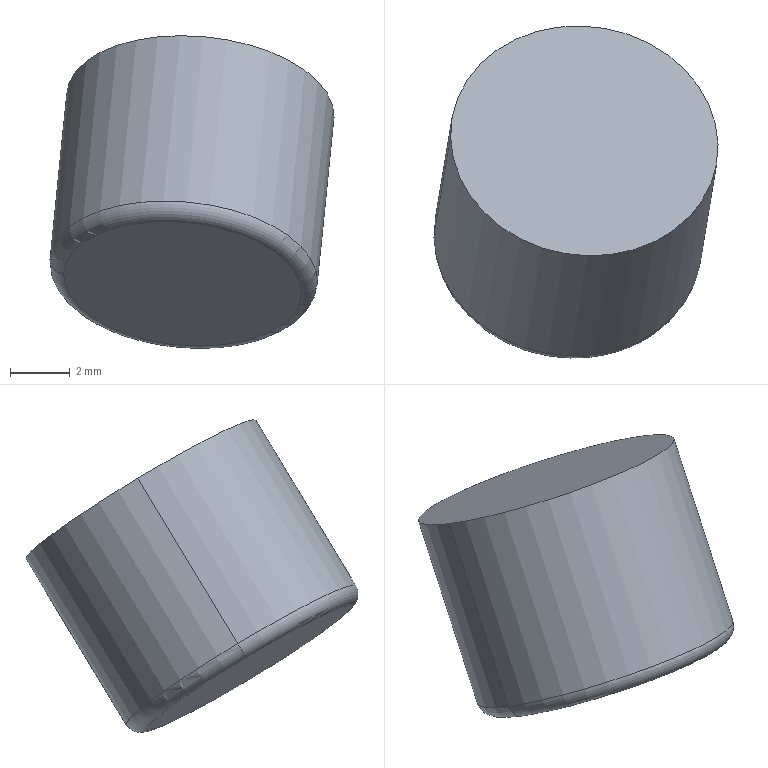Component | SolidWorks | 14AC-24-1-015-1 | 1 solid | 6 faces | box 9.53 x 11.13 x 10.48 mm | volume 444 mm3 | torus 2 | cylinder 2 | plane 2 | commonest cylinder face diameters 9 x2
build123d program:
from build123d import *

# Parameters (mm, degrees)
SKETCH1_R           = 4.5
BOSS_EXTRUDE1_DEPTH = 7
FILLET1_R           = 0.5


with BuildPart() as part:
    # Sketch1 → Boss-Extrude1 (new body)
    with BuildSketch(Plane.XY):
        Circle(SKETCH1_R)
    extrude(amount=BOSS_EXTRUDE1_DEPTH)

    # Fillet1
    fillet1_edges = [part.edges().sort_by_distance(p)[0] for p in [
        (-4.5, 0, 0),
    ]]
    fillet(fillet1_edges, radius=FILLET1_R)


solid = part.part

# Placed as in the assembly
solid = solid.moved(Location((420.449, -136.308, -150.512), (-31.129, 4.92, 15.941)))
STEP:
#1=COLOUR_RGB('',0.7922,0.8196,0.9333);
#2=FILL_AREA_STYLE_COLOUR('',#1);
#3=FILL_AREA_STYLE('',(#2));
#4=SURFACE_STYLE_FILL_AREA(#3);
#5=SURFACE_SIDE_STYLE('',(#4));
#6=SURFACE_STYLE_USAGE(.BOTH.,#5);
#7=PRESENTATION_STYLE_ASSIGNMENT((#6));
#8=CARTESIAN_POINT('',(16.396,-5.363,-5.912));
#9=VERTEX_POINT('',#8);
#10=CARTESIAN_POINT('',(16.71,-5.37,-5.939));
#11=VERTEX_POINT('',#10);
#12=CARTESIAN_POINT('',(16.553,-5.366,-5.926));
#13=DIRECTION('',(-0.08576,-0.5151,-0.8529));
#14=DIRECTION('',(0.996,-0.02384,-0.08576));
#15=AXIS2_PLACEMENT_3D('',#12,#13,#14);
#16=CIRCLE('',#15,0.1575);
#17=EDGE_CURVE('',#9,#11,#16,.T.);
#18=ORIENTED_EDGE('',*,*,#17,.F.);
#19=CARTESIAN_POINT('',(16.378,-5.352,-5.894));
#20=VERTEX_POINT('',#19);
#21=CARTESIAN_POINT('',(16.398,-5.353,-5.895));
#22=DIRECTION('',(-0.02384,0.8568,-0.5151));
#23=DIRECTION('',(0.,0.5152,0.8571));
#24=AXIS2_PLACEMENT_3D('',#21,#22,#23);
#25=CIRCLE('',#24,0.01969);
#26=EDGE_CURVE('',#9,#20,#25,.T.);
#27=ORIENTED_EDGE('',*,*,#26,.T.);
#28=CARTESIAN_POINT('',(16.731,-5.361,-5.924));
#29=VERTEX_POINT('',#28);
#30=CARTESIAN_POINT('',(16.555,-5.356,-5.909));
#31=DIRECTION('',(0.08576,0.5151,0.8529));
#32=DIRECTION('',(0.996,-0.02384,-0.08576));
#33=AXIS2_PLACEMENT_3D('',#30,#31,#32);
#34=CIRCLE('',#33,0.1772);
#35=EDGE_CURVE('',#29,#20,#34,.T.);
#36=ORIENTED_EDGE('',*,*,#35,.F.);
#37=CARTESIAN_POINT('',(16.712,-5.36,-5.922));
#38=DIRECTION('',(0.02384,-0.8568,0.5151));
#39=DIRECTION('',(0.,-0.5152,-0.8571));
#40=AXIS2_PLACEMENT_3D('',#37,#38,#39);
#41=CIRCLE('',#40,0.01969);
#42=EDGE_CURVE('',#11,#29,#41,.T.);
#43=ORIENTED_EDGE('',*,*,#42,.F.);
#44=EDGE_LOOP('',(#18,#27,#36,#43));
#45=FACE_OUTER_BOUND('',#44,.T.);
#46=CARTESIAN_POINT('',(16.555,-5.356,-5.909));
#47=DIRECTION('',(0.08576,0.5151,0.8529));
#48=DIRECTION('',(0.996,-0.02384,-0.08576));
#49=AXIS2_PLACEMENT_3D('',#46,#47,#48);
#50=TOROIDAL_SURFACE('',#49,0.1575,0.01969);
#51=ADVANCED_FACE('',(#45),#50,.T.);
#52=CARTESIAN_POINT('',(16.753,-5.229,-5.706));
#53=VERTEX_POINT('',#52);
#54=CARTESIAN_POINT('',(16.4,-5.22,-5.675));
#55=VERTEX_POINT('',#54);
#56=CARTESIAN_POINT('',(16.577,-5.224,-5.691));
#57=DIRECTION('',(0.08576,0.5151,0.8529));
#58=DIRECTION('',(0.996,-0.02384,-0.08576));
#59=AXIS2_PLACEMENT_3D('',#56,#57,#58);
#60=CIRCLE('',#59,0.1772);
#61=EDGE_CURVE('',#53,#55,#60,.T.);
#62=ORIENTED_EDGE('',*,*,#61,.F.);
#63=CARTESIAN_POINT('',(16.753,-5.229,-5.706));
#64=DIRECTION('',(-0.08576,-0.5151,-0.8529));
#65=VECTOR('',#64,39.37);
#66=LINE('',#63,#65);
#67=EDGE_CURVE('',#53,#29,#66,.T.);
#68=ORIENTED_EDGE('',*,*,#67,.T.);
#69=ORIENTED_EDGE('',*,*,#35,.T.);
#70=CARTESIAN_POINT('',(16.4,-5.22,-5.675));
#71=DIRECTION('',(-0.08576,-0.5151,-0.8529));
#72=VECTOR('',#71,39.37);
#73=LINE('',#70,#72);
#74=EDGE_CURVE('',#55,#20,#73,.T.);
#75=ORIENTED_EDGE('',*,*,#74,.F.);
#76=EDGE_LOOP('',(#62,#68,#69,#75));
#77=FACE_OUTER_BOUND('',#76,.T.);
#78=CARTESIAN_POINT('',(16.577,-5.224,-5.691));
#79=DIRECTION('',(-0.08576,-0.5151,-0.8529));
#80=DIRECTION('',(-0.996,0.02384,0.08576));
#81=AXIS2_PLACEMENT_3D('',#78,#79,#80);
#82=CYLINDRICAL_SURFACE('',#81,0.1772);
#83=ADVANCED_FACE('',(#77),#82,.T.);
#84=ORIENTED_EDGE('',*,*,#67,.F.);
#85=CARTESIAN_POINT('',(16.577,-5.224,-5.691));
#86=DIRECTION('',(0.08576,0.5151,0.8529));
#87=DIRECTION('',(0.996,-0.02384,-0.08576));
#88=AXIS2_PLACEMENT_3D('',#85,#86,#87);
#89=CIRCLE('',#88,0.1772);
#90=EDGE_CURVE('',#55,#53,#89,.T.);
#91=ORIENTED_EDGE('',*,*,#90,.F.);
#92=ORIENTED_EDGE('',*,*,#74,.T.);
#93=CARTESIAN_POINT('',(16.555,-5.356,-5.909));
#94=DIRECTION('',(0.08576,0.5151,0.8529));
#95=DIRECTION('',(0.996,-0.02384,-0.08576));
#96=AXIS2_PLACEMENT_3D('',#93,#94,#95);
#97=CIRCLE('',#96,0.1772);
#98=EDGE_CURVE('',#20,#29,#97,.T.);
#99=ORIENTED_EDGE('',*,*,#98,.T.);
#100=EDGE_LOOP('',(#84,#91,#92,#99));
#101=FACE_OUTER_BOUND('',#100,.T.);
#102=CARTESIAN_POINT('',(16.577,-5.224,-5.691));
#103=DIRECTION('',(-0.08576,-0.5151,-0.8529));
#104=DIRECTION('',(-0.996,0.02384,0.08576));
#105=AXIS2_PLACEMENT_3D('',#102,#103,#104);
#106=CYLINDRICAL_SURFACE('',#105,0.1772);
#107=ADVANCED_FACE('',(#101),#106,.T.);
#108=ORIENTED_EDGE('',*,*,#90,.T.);
#109=ORIENTED_EDGE('',*,*,#61,.T.);
#110=EDGE_LOOP('',(#108,#109));
#111=FACE_OUTER_BOUND('',#110,.T.);
#112=CARTESIAN_POINT('',(16.577,-5.224,-5.691));
#113=DIRECTION('',(0.08576,0.5151,0.8529));
#114=DIRECTION('',(0.996,-0.02384,-0.08576));
#115=AXIS2_PLACEMENT_3D('',#112,#113,#114);
#116=PLANE('',#115);
#117=ADVANCED_FACE('',(#111),#116,.T.);
#118=CARTESIAN_POINT('',(16.553,-5.366,-5.926));
#119=DIRECTION('',(-0.08576,-0.5151,-0.8529));
#120=DIRECTION('',(0.996,-0.02384,-0.08576));
#121=AXIS2_PLACEMENT_3D('',#118,#119,#120);
#122=CIRCLE('',#121,0.1575);
#123=EDGE_CURVE('',#11,#9,#122,.T.);
#124=ORIENTED_EDGE('',*,*,#123,.T.);
#125=ORIENTED_EDGE('',*,*,#17,.T.);
#126=EDGE_LOOP('',(#124,#125));
#127=FACE_OUTER_BOUND('',#126,.T.);
#128=CARTESIAN_POINT('',(16.553,-5.366,-5.926));
#129=DIRECTION('',(0.08576,0.5151,0.8529));
#130=DIRECTION('',(0.996,-0.02384,-0.08576));
#131=AXIS2_PLACEMENT_3D('',#128,#129,#130);
#132=PLANE('',#131);
#133=ADVANCED_FACE('',(#127),#132,.F.);
#134=ORIENTED_EDGE('',*,*,#26,.F.);
#135=ORIENTED_EDGE('',*,*,#123,.F.);
#136=ORIENTED_EDGE('',*,*,#42,.T.);
#137=ORIENTED_EDGE('',*,*,#98,.F.);
#138=EDGE_LOOP('',(#134,#135,#136,#137));
#139=FACE_OUTER_BOUND('',#138,.T.);
#140=CARTESIAN_POINT('',(16.555,-5.356,-5.909));
#141=DIRECTION('',(0.08576,0.5151,0.8529));
#142=DIRECTION('',(0.996,-0.02384,-0.08576));
#143=AXIS2_PLACEMENT_3D('',#140,#141,#142);
#144=TOROIDAL_SURFACE('',#143,0.1575,0.01969);
#145=ADVANCED_FACE('',(#139),#144,.T.);
#146=CLOSED_SHELL('',(#51,#83,#107,#117,#133,#145));
#147=MANIFOLD_SOLID_BREP('',#146);
#148=STYLED_ITEM('',(#7),#147);
#149=(LENGTH_UNIT()NAMED_UNIT(*)SI_UNIT($,.METRE.));
#150=LENGTH_MEASURE_WITH_UNIT(LENGTH_MEASURE(0.0254),#149);
#151=DIMENSIONAL_EXPONENTS(1.,0.,0.,0.,0.,0.,0.);
#152=(CONVERSION_BASED_UNIT('',#150)LENGTH_UNIT()NAMED_UNIT(#151));
#153=UNCERTAINTY_MEASURE_WITH_UNIT(LENGTH_MEASURE(0.00001),#152,'','');
#154=(NAMED_UNIT(*)PLANE_ANGLE_UNIT()SI_UNIT($,.RADIAN.));
#155=(NAMED_UNIT(*)SI_UNIT($,.STERADIAN.)SOLID_ANGLE_UNIT());
#156=(GEOMETRIC_REPRESENTATION_CONTEXT(3)GLOBAL_UNCERTAINTY_ASSIGNED_CONTEXT((#153))GLOBAL_UNIT_ASSIGNED_CONTEXT((#152,#154,#155))REPRESENTATION_CONTEXT('',''));
#157=MECHANICAL_DESIGN_GEOMETRIC_PRESENTATION_REPRESENTATION('',(#148),#156);
#158=PRESENTATION_LAYER_ASSIGNMENT('','',(#148));
#159=CARTESIAN_POINT('',(0.,0.,0.));
#160=DIRECTION('',(0.,0.,1.));
#161=DIRECTION('',(1.,0.,0.));
#162=AXIS2_PLACEMENT_3D('',#159,#160,#161);
#163=(LENGTH_UNIT()NAMED_UNIT(*)SI_UNIT($,.METRE.));
#164=LENGTH_MEASURE_WITH_UNIT(LENGTH_MEASURE(0.0254),#163);
#165=DIMENSIONAL_EXPONENTS(1.,0.,0.,0.,0.,0.,0.);
#166=(CONVERSION_BASED_UNIT('',#164)LENGTH_UNIT()NAMED_UNIT(#165));
#167=UNCERTAINTY_MEASURE_WITH_UNIT(LENGTH_MEASURE(0.00001),#166,'','');
#168=(NAMED_UNIT(*)PLANE_ANGLE_UNIT()SI_UNIT($,.RADIAN.));
#169=(NAMED_UNIT(*)SI_UNIT($,.STERADIAN.)SOLID_ANGLE_UNIT());
#170=(GEOMETRIC_REPRESENTATION_CONTEXT(3)GLOBAL_UNCERTAINTY_ASSIGNED_CONTEXT((#167))GLOBAL_UNIT_ASSIGNED_CONTEXT((#166,#168,#169))REPRESENTATION_CONTEXT('',''));
#171=ADVANCED_BREP_SHAPE_REPRESENTATION('',(#147,#162),#170);